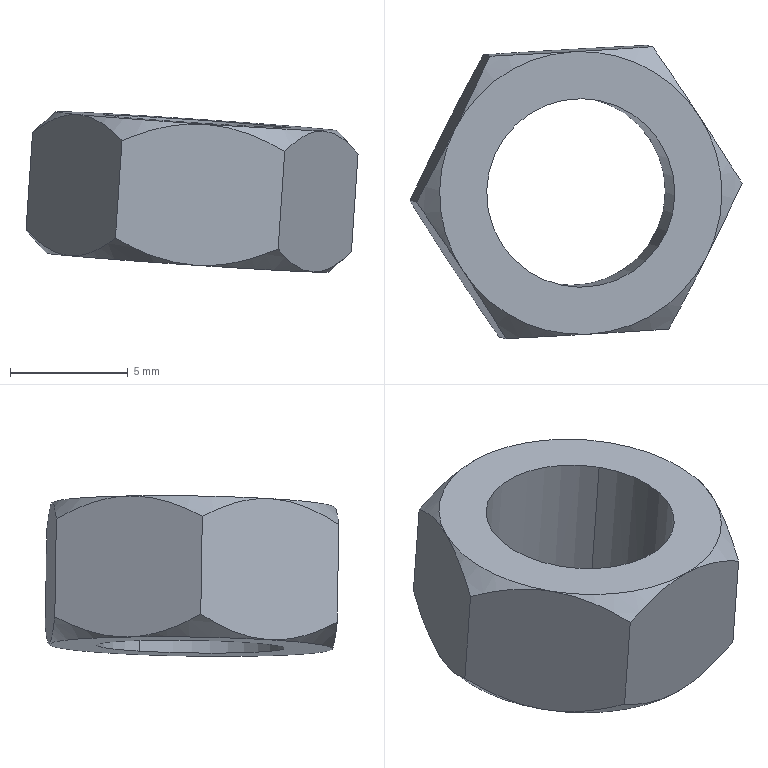Component | SolidWorks | SDAJ25x20-20B(00)+()-1_SDAJ-25- M8x1_25-1 | 1 solid | 22 faces | box 14.08 x 12.45 x 6.82 mm | volume 440 mm3 | cone 12 | plane 8 | cylinder 2 | commonest cylinder face diameters 8 x2
STEP:
#1=CARTESIAN_POINT('',(-3.493,5.702,30.763));
#2=VERTEX_POINT('',#1);
#3=CARTESIAN_POINT('',(-3.756,5.529,30.778));
#4=VERTEX_POINT('',#3);
#5=CARTESIAN_POINT('',(-3.493,5.702,30.763));
#6=CARTESIAN_POINT('',(-3.482,5.685,30.762));
#7=CARTESIAN_POINT('',(-3.474,5.666,30.761));
#8=CARTESIAN_POINT('',(-3.467,5.625,30.76));
#9=CARTESIAN_POINT('',(-3.467,5.604,30.76));
#10=CARTESIAN_POINT('',(-3.475,5.564,30.76));
#11=CARTESIAN_POINT('',(-3.483,5.544,30.76));
#12=CARTESIAN_POINT('',(-3.506,5.51,30.761));
#13=CARTESIAN_POINT('',(-3.521,5.495,30.762));
#14=CARTESIAN_POINT('',(-3.556,5.473,30.764));
#15=CARTESIAN_POINT('',(-3.575,5.465,30.765));
#16=CARTESIAN_POINT('',(-3.616,5.457,30.768));
#17=CARTESIAN_POINT('',(-3.636,5.457,30.769));
#18=CARTESIAN_POINT('',(-3.677,5.466,30.772));
#19=CARTESIAN_POINT('',(-3.696,5.474,30.773));
#20=CARTESIAN_POINT('',(-3.73,5.497,30.776));
#21=CARTESIAN_POINT('',(-3.745,5.512,30.777));
#22=CARTESIAN_POINT('',(-3.756,5.529,30.778));
#23=B_SPLINE_CURVE_WITH_KNOTS('',3,(#5,#6,#7,#8,#9,#10,#11,#12,#13,#14,#15,#16,#17,#18,#19,#20,#21,#22),.UNSPECIFIED.,.F.,.F.,(4,2,2,2,2,2,2,2,4),(0.,0.0625,0.125,0.1875,0.25,0.3125,0.375,0.4375,0.5),.UNSPECIFIED.);
#24=EDGE_CURVE('',#2,#4,#23,.T.);
#25=ORIENTED_EDGE('',*,*,#24,.F.);
#26=CARTESIAN_POINT('',(-3.509,5.706,30.527));
#27=VERTEX_POINT('',#26);
#28=CARTESIAN_POINT('',(-3.493,5.702,30.763));
#29=DIRECTION('',(-0.0675,0.01553,-0.9976));
#30=VECTOR('',#29,39.37);
#31=LINE('',#28,#30);
#32=EDGE_CURVE('',#2,#27,#31,.T.);
#33=ORIENTED_EDGE('',*,*,#32,.T.);
#34=CARTESIAN_POINT('',(-3.772,5.533,30.543));
#35=VERTEX_POINT('',#34);
#36=CARTESIAN_POINT('',(-3.641,5.619,30.535));
#37=DIRECTION('',(-0.0675,0.01553,-0.9976));
#38=DIRECTION('',(-0.8341,-0.5496,0.04788));
#39=AXIS2_PLACEMENT_3D('',#36,#37,#38);
#40=CIRCLE('',#39,0.1575);
#41=EDGE_CURVE('',#27,#35,#40,.T.);
#42=ORIENTED_EDGE('',*,*,#41,.T.);
#43=CARTESIAN_POINT('',(-3.756,5.529,30.778));
#44=DIRECTION('',(-0.0675,0.01553,-0.9976));
#45=VECTOR('',#44,39.37);
#46=LINE('',#43,#45);
#47=EDGE_CURVE('',#4,#35,#46,.T.);
#48=ORIENTED_EDGE('',*,*,#47,.F.);
#49=EDGE_LOOP('',(#25,#33,#42,#48));
#50=FACE_OUTER_BOUND('',#49,.T.);
#51=CARTESIAN_POINT('',(-3.625,5.616,30.771));
#52=DIRECTION('',(-0.0675,0.01553,-0.9976));
#53=DIRECTION('',(-0.8341,-0.5496,0.04788));
#54=AXIS2_PLACEMENT_3D('',#51,#52,#53);
#55=CYLINDRICAL_SURFACE('',#54,0.1575);
#56=ADVANCED_FACE('',(#50),#55,.F.);
#57=CARTESIAN_POINT('',(-3.611,5.38,30.766));
#58=VERTEX_POINT('',#57);
#59=CARTESIAN_POINT('',(-3.478,5.388,30.721));
#60=VERTEX_POINT('',#59);
#61=CARTESIAN_POINT('',(-3.611,5.38,30.766));
#62=CARTESIAN_POINT('',(-3.588,5.381,30.764));
#63=CARTESIAN_POINT('',(-3.565,5.383,30.759));
#64=CARTESIAN_POINT('',(-3.52,5.386,30.743));
#65=CARTESIAN_POINT('',(-3.498,5.387,30.733));
#66=CARTESIAN_POINT('',(-3.478,5.388,30.721));
#67=B_SPLINE_CURVE_WITH_KNOTS('',3,(#61,#62,#63,#64,#65,#66),.UNSPECIFIED.,.F.,.F.,(4,2,4),(0.003591,0.005374,0.007157),.UNSPECIFIED.);
#68=EDGE_CURVE('',#58,#60,#67,.T.);
#69=ORIENTED_EDGE('',*,*,#68,.T.);
#70=CARTESIAN_POINT('',(-3.414,5.51,30.755));
#71=VERTEX_POINT('',#70);
#72=CARTESIAN_POINT('',(-3.478,5.388,30.721));
#73=CARTESIAN_POINT('',(-3.468,5.407,30.731));
#74=CARTESIAN_POINT('',(-3.457,5.427,30.74));
#75=CARTESIAN_POINT('',(-3.441,5.457,30.749));
#76=CARTESIAN_POINT('',(-3.436,5.467,30.751));
#77=CARTESIAN_POINT('',(-3.425,5.488,30.754));
#78=CARTESIAN_POINT('',(-3.42,5.499,30.755));
#79=CARTESIAN_POINT('',(-3.414,5.51,30.755));
#80=B_SPLINE_CURVE_WITH_KNOTS('',3,(#72,#73,#74,#75,#76,#77,#78,#79),.UNSPECIFIED.,.F.,.F.,(4,2,2,4),(0.00000025,0.001796,0.002693,0.003591),.UNSPECIFIED.);
#81=EDGE_CURVE('',#60,#71,#80,.T.);
#82=ORIENTED_EDGE('',*,*,#81,.T.);
#83=CARTESIAN_POINT('',(-3.625,5.616,30.771));
#84=DIRECTION('',(0.0675,-0.01553,0.9976));
#85=DIRECTION('',(0.8341,0.5496,-0.04788));
#86=AXIS2_PLACEMENT_3D('',#83,#84,#85);
#87=CIRCLE('',#86,0.2362);
#88=EDGE_CURVE('',#58,#71,#87,.T.);
#89=ORIENTED_EDGE('',*,*,#88,.F.);
#90=EDGE_LOOP('',(#69,#82,#89));
#91=FACE_OUTER_BOUND('',#90,.T.);
#92=CARTESIAN_POINT('',(-3.628,5.616,30.724));
#93=DIRECTION('',(-0.0675,0.01553,-0.9976));
#94=DIRECTION('',(-0.8341,-0.5496,0.04788));
#95=AXIS2_PLACEMENT_3D('',#92,#93,#94);
#96=CONICAL_SURFACE('',#95,0.2835,0.7854);
#97=ADVANCED_FACE('',(#91),#96,.T.);
#98=CARTESIAN_POINT('',(-3.428,5.745,30.759));
#99=VERTEX_POINT('',#98);
#100=CARTESIAN_POINT('',(-3.625,5.616,30.771));
#101=DIRECTION('',(0.0675,-0.01553,0.9976));
#102=DIRECTION('',(0.8341,0.5496,-0.04788));
#103=AXIS2_PLACEMENT_3D('',#100,#101,#102);
#104=CIRCLE('',#103,0.2362);
#105=EDGE_CURVE('',#71,#99,#104,.T.);
#106=ORIENTED_EDGE('',*,*,#105,.F.);
#107=CARTESIAN_POINT('',(-3.355,5.632,30.716));
#108=VERTEX_POINT('',#107);
#109=CARTESIAN_POINT('',(-3.414,5.51,30.755));
#110=CARTESIAN_POINT('',(-3.404,5.531,30.754));
#111=CARTESIAN_POINT('',(-3.393,5.552,30.75));
#112=CARTESIAN_POINT('',(-3.374,5.593,30.737));
#113=CARTESIAN_POINT('',(-3.364,5.613,30.727));
#114=CARTESIAN_POINT('',(-3.355,5.632,30.716));
#115=B_SPLINE_CURVE_WITH_KNOTS('',3,(#109,#110,#111,#112,#113,#114),.UNSPECIFIED.,.F.,.F.,(4,2,4),(0.003591,0.005374,0.007157),.UNSPECIFIED.);
#116=EDGE_CURVE('',#71,#108,#115,.T.);
#117=ORIENTED_EDGE('',*,*,#116,.T.);
#118=CARTESIAN_POINT('',(-3.355,5.632,30.716));
#119=CARTESIAN_POINT('',(-3.366,5.65,30.728));
#120=CARTESIAN_POINT('',(-3.378,5.668,30.738));
#121=CARTESIAN_POINT('',(-3.396,5.696,30.749));
#122=CARTESIAN_POINT('',(-3.402,5.706,30.753));
#123=CARTESIAN_POINT('',(-3.415,5.726,30.757));
#124=CARTESIAN_POINT('',(-3.421,5.735,30.759));
#125=CARTESIAN_POINT('',(-3.428,5.745,30.759));
#126=B_SPLINE_CURVE_WITH_KNOTS('',3,(#118,#119,#120,#121,#122,#123,#124,#125),.UNSPECIFIED.,.F.,.F.,(4,2,2,4),(0.004638,0.006433,0.007331,0.008228),.UNSPECIFIED.);
#127=EDGE_CURVE('',#108,#99,#126,.T.);
#128=ORIENTED_EDGE('',*,*,#127,.T.);
#129=EDGE_LOOP('',(#106,#117,#128));
#130=FACE_OUTER_BOUND('',#129,.T.);
#131=CARTESIAN_POINT('',(-3.628,5.616,30.724));
#132=DIRECTION('',(-0.0675,0.01553,-0.9976));
#133=DIRECTION('',(-0.8341,-0.5496,0.04788));
#134=AXIS2_PLACEMENT_3D('',#131,#132,#133);
#135=CONICAL_SURFACE('',#134,0.2835,0.7854);
#136=ADVANCED_FACE('',(#130),#135,.T.);
#137=CARTESIAN_POINT('',(-3.638,5.851,30.775));
#138=VERTEX_POINT('',#137);
#139=CARTESIAN_POINT('',(-3.625,5.616,30.771));
#140=DIRECTION('',(0.0675,-0.01553,0.9976));
#141=DIRECTION('',(0.8341,0.5496,-0.04788));
#142=AXIS2_PLACEMENT_3D('',#139,#140,#141);
#143=CIRCLE('',#142,0.2362);
#144=EDGE_CURVE('',#99,#138,#143,.T.);
#145=ORIENTED_EDGE('',*,*,#144,.F.);
#146=CARTESIAN_POINT('',(-3.505,5.86,30.73));
#147=VERTEX_POINT('',#146);
#148=CARTESIAN_POINT('',(-3.428,5.745,30.759));
#149=CARTESIAN_POINT('',(-3.441,5.766,30.761));
#150=CARTESIAN_POINT('',(-3.454,5.785,30.758));
#151=CARTESIAN_POINT('',(-3.473,5.814,30.75));
#152=CARTESIAN_POINT('',(-3.48,5.823,30.747));
#153=CARTESIAN_POINT('',(-3.492,5.842,30.739));
#154=CARTESIAN_POINT('',(-3.499,5.851,30.734));
#155=CARTESIAN_POINT('',(-3.505,5.86,30.73));
#156=B_SPLINE_CURVE_WITH_KNOTS('',3,(#148,#149,#150,#151,#152,#153,#154,#155),.UNSPECIFIED.,.F.,.F.,(4,2,2,4),(0.008228,0.01003,0.01092,0.01182),.UNSPECIFIED.);
#157=EDGE_CURVE('',#99,#147,#156,.T.);
#158=ORIENTED_EDGE('',*,*,#157,.T.);
#159=CARTESIAN_POINT('',(-3.505,5.86,30.73));
#160=CARTESIAN_POINT('',(-3.525,5.859,30.742));
#161=CARTESIAN_POINT('',(-3.547,5.857,30.752));
#162=CARTESIAN_POINT('',(-3.58,5.855,30.764));
#163=CARTESIAN_POINT('',(-3.591,5.854,30.768));
#164=CARTESIAN_POINT('',(-3.614,5.853,30.773));
#165=CARTESIAN_POINT('',(-3.626,5.852,30.774));
#166=CARTESIAN_POINT('',(-3.638,5.851,30.775));
#167=B_SPLINE_CURVE_WITH_KNOTS('',3,(#159,#160,#161,#162,#163,#164,#165,#166),.UNSPECIFIED.,.F.,.F.,(4,2,2,4),(0.00000025,0.001796,0.002693,0.003591),.UNSPECIFIED.);
#168=EDGE_CURVE('',#147,#138,#167,.T.);
#169=ORIENTED_EDGE('',*,*,#168,.T.);
#170=EDGE_LOOP('',(#145,#158,#169));
#171=FACE_OUTER_BOUND('',#170,.T.);
#172=CARTESIAN_POINT('',(-3.628,5.616,30.724));
#173=DIRECTION('',(-0.0675,0.01553,-0.9976));
#174=DIRECTION('',(-0.8341,-0.5496,0.04788));
#175=AXIS2_PLACEMENT_3D('',#172,#173,#174);
#176=CONICAL_SURFACE('',#175,0.2835,0.7854);
#177=ADVANCED_FACE('',(#171),#176,.T.);
#178=CARTESIAN_POINT('',(-3.822,5.486,30.782));
#179=VERTEX_POINT('',#178);
#180=CARTESIAN_POINT('',(-3.75,5.372,30.739));
#181=VERTEX_POINT('',#180);
#182=CARTESIAN_POINT('',(-3.822,5.486,30.782));
#183=CARTESIAN_POINT('',(-3.815,5.476,30.781));
#184=CARTESIAN_POINT('',(-3.809,5.466,30.78));
#185=CARTESIAN_POINT('',(-3.796,5.446,30.775));
#186=CARTESIAN_POINT('',(-3.79,5.437,30.772));
#187=CARTESIAN_POINT('',(-3.772,5.408,30.761));
#188=CARTESIAN_POINT('',(-3.76,5.39,30.75));
#189=CARTESIAN_POINT('',(-3.75,5.372,30.739));
#190=B_SPLINE_CURVE_WITH_KNOTS('',3,(#182,#183,#184,#185,#186,#187,#188,#189),.UNSPECIFIED.,.F.,.F.,(4,2,2,4),(0.007255,0.008152,0.009049,0.01084),.UNSPECIFIED.);
#191=EDGE_CURVE('',#179,#181,#190,.T.);
#192=ORIENTED_EDGE('',*,*,#191,.T.);
#193=CARTESIAN_POINT('',(-3.75,5.372,30.739));
#194=CARTESIAN_POINT('',(-3.728,5.374,30.748));
#195=CARTESIAN_POINT('',(-3.705,5.375,30.756));
#196=CARTESIAN_POINT('',(-3.671,5.377,30.763));
#197=CARTESIAN_POINT('',(-3.659,5.377,30.765));
#198=CARTESIAN_POINT('',(-3.635,5.378,30.767));
#199=CARTESIAN_POINT('',(-3.623,5.379,30.767));
#200=CARTESIAN_POINT('',(-3.611,5.38,30.766));
#201=B_SPLINE_CURVE_WITH_KNOTS('',3,(#193,#194,#195,#196,#197,#198,#199,#200),.UNSPECIFIED.,.F.,.F.,(4,2,2,4),(0.00000025,0.001796,0.002693,0.003591),.UNSPECIFIED.);
#202=EDGE_CURVE('',#181,#58,#201,.T.);
#203=ORIENTED_EDGE('',*,*,#202,.T.);
#204=CARTESIAN_POINT('',(-3.625,5.616,30.771));
#205=DIRECTION('',(0.0675,-0.01553,0.9976));
#206=DIRECTION('',(0.8341,0.5496,-0.04788));
#207=AXIS2_PLACEMENT_3D('',#204,#205,#206);
#208=CIRCLE('',#207,0.2362);
#209=EDGE_CURVE('',#179,#58,#208,.T.);
#210=ORIENTED_EDGE('',*,*,#209,.F.);
#211=EDGE_LOOP('',(#192,#203,#210));
#212=FACE_OUTER_BOUND('',#211,.T.);
#213=CARTESIAN_POINT('',(-3.628,5.616,30.724));
#214=DIRECTION('',(-0.0675,0.01553,-0.9976));
#215=DIRECTION('',(-0.8341,-0.5496,0.04788));
#216=AXIS2_PLACEMENT_3D('',#213,#214,#215);
#217=CONICAL_SURFACE('',#216,0.2835,0.7854);
#218=ADVANCED_FACE('',(#212),#217,.T.);
#219=CARTESIAN_POINT('',(-3.835,5.722,30.787));
#220=VERTEX_POINT('',#219);
#221=CARTESIAN_POINT('',(-3.625,5.616,30.771));
#222=DIRECTION('',(0.0675,-0.01553,0.9976));
#223=DIRECTION('',(0.8341,0.5496,-0.04788));
#224=AXIS2_PLACEMENT_3D('',#221,#222,#223);
#225=CIRCLE('',#224,0.2362);
#226=EDGE_CURVE('',#138,#220,#225,.T.);
#227=ORIENTED_EDGE('',*,*,#226,.F.);
#228=CARTESIAN_POINT('',(-3.777,5.844,30.748));
#229=VERTEX_POINT('',#228);
#230=CARTESIAN_POINT('',(-3.638,5.851,30.775));
#231=CARTESIAN_POINT('',(-3.662,5.85,30.777));
#232=CARTESIAN_POINT('',(-3.685,5.849,30.775));
#233=CARTESIAN_POINT('',(-3.732,5.846,30.765));
#234=CARTESIAN_POINT('',(-3.755,5.845,30.757));
#235=CARTESIAN_POINT('',(-3.777,5.844,30.748));
#236=B_SPLINE_CURVE_WITH_KNOTS('',3,(#230,#231,#232,#233,#234,#235),.UNSPECIFIED.,.F.,.F.,(4,2,4),(0.003591,0.005374,0.007157),.UNSPECIFIED.);
#237=EDGE_CURVE('',#138,#229,#236,.T.);
#238=ORIENTED_EDGE('',*,*,#237,.T.);
#239=CARTESIAN_POINT('',(-3.777,5.844,30.748));
#240=CARTESIAN_POINT('',(-3.785,5.825,30.759));
#241=CARTESIAN_POINT('',(-3.795,5.805,30.768));
#242=CARTESIAN_POINT('',(-3.809,5.775,30.779));
#243=CARTESIAN_POINT('',(-3.814,5.764,30.781));
#244=CARTESIAN_POINT('',(-3.824,5.743,30.785));
#245=CARTESIAN_POINT('',(-3.83,5.732,30.786));
#246=CARTESIAN_POINT('',(-3.835,5.722,30.787));
#247=B_SPLINE_CURVE_WITH_KNOTS('',3,(#239,#240,#241,#242,#243,#244,#245,#246),.UNSPECIFIED.,.F.,.F.,(4,2,2,4),(0.00000025,0.001796,0.002693,0.003591),.UNSPECIFIED.);
#248=EDGE_CURVE('',#229,#220,#247,.T.);
#249=ORIENTED_EDGE('',*,*,#248,.T.);
#250=EDGE_LOOP('',(#227,#238,#249));
#251=FACE_OUTER_BOUND('',#250,.T.);
#252=CARTESIAN_POINT('',(-3.628,5.616,30.724));
#253=DIRECTION('',(-0.0675,0.01553,-0.9976));
#254=DIRECTION('',(-0.8341,-0.5496,0.04788));
#255=AXIS2_PLACEMENT_3D('',#252,#253,#254);
#256=CONICAL_SURFACE('',#255,0.2835,0.7854);
#257=ADVANCED_FACE('',(#251),#256,.T.);
#258=CARTESIAN_POINT('',(-3.851,5.725,30.551));
#259=VERTEX_POINT('',#258);
#260=CARTESIAN_POINT('',(-3.788,5.847,30.585));
#261=VERTEX_POINT('',#260);
#262=CARTESIAN_POINT('',(-3.851,5.725,30.551));
#263=CARTESIAN_POINT('',(-3.841,5.747,30.55));
#264=CARTESIAN_POINT('',(-3.83,5.767,30.554));
#265=CARTESIAN_POINT('',(-3.808,5.808,30.566));
#266=CARTESIAN_POINT('',(-3.798,5.828,30.575));
#267=CARTESIAN_POINT('',(-3.788,5.847,30.585));
#268=B_SPLINE_CURVE_WITH_KNOTS('',3,(#262,#263,#264,#265,#266,#267),.UNSPECIFIED.,.F.,.F.,(4,2,4),(0.003591,0.005374,0.007157),.UNSPECIFIED.);
#269=EDGE_CURVE('',#259,#261,#268,.T.);
#270=ORIENTED_EDGE('',*,*,#269,.T.);
#271=CARTESIAN_POINT('',(-3.654,5.855,30.54));
#272=VERTEX_POINT('',#271);
#273=CARTESIAN_POINT('',(-3.788,5.847,30.585));
#274=CARTESIAN_POINT('',(-3.767,5.848,30.573));
#275=CARTESIAN_POINT('',(-3.746,5.849,30.562));
#276=CARTESIAN_POINT('',(-3.713,5.852,30.551));
#277=CARTESIAN_POINT('',(-3.701,5.852,30.547));
#278=CARTESIAN_POINT('',(-3.678,5.854,30.542));
#279=CARTESIAN_POINT('',(-3.666,5.854,30.54));
#280=CARTESIAN_POINT('',(-3.654,5.855,30.54));
#281=B_SPLINE_CURVE_WITH_KNOTS('',3,(#273,#274,#275,#276,#277,#278,#279,#280),.UNSPECIFIED.,.F.,.F.,(4,2,2,4),(0.00000025,0.001796,0.002693,0.003591),.UNSPECIFIED.);
#282=EDGE_CURVE('',#261,#272,#281,.T.);
#283=ORIENTED_EDGE('',*,*,#282,.T.);
#284=CARTESIAN_POINT('',(-3.641,5.619,30.535));
#285=DIRECTION('',(0.0675,-0.01553,0.9976));
#286=DIRECTION('',(0.8341,0.5496,-0.04788));
#287=AXIS2_PLACEMENT_3D('',#284,#285,#286);
#288=CIRCLE('',#287,0.2362);
#289=EDGE_CURVE('',#272,#259,#288,.T.);
#290=ORIENTED_EDGE('',*,*,#289,.T.);
#291=EDGE_LOOP('',(#270,#283,#290));
#292=FACE_OUTER_BOUND('',#291,.T.);
#293=CARTESIAN_POINT('',(-3.641,5.619,30.535));
#294=DIRECTION('',(0.0675,-0.01553,0.9976));
#295=DIRECTION('',(0.8341,0.5496,-0.04788));
#296=AXIS2_PLACEMENT_3D('',#293,#294,#295);
#297=CONICAL_SURFACE('',#296,0.2362,0.7854);
#298=ADVANCED_FACE('',(#292),#297,.T.);
#299=CARTESIAN_POINT('',(-3.444,5.749,30.524));
#300=VERTEX_POINT('',#299);
#301=CARTESIAN_POINT('',(-3.641,5.619,30.535));
#302=DIRECTION('',(0.0675,-0.01553,0.9976));
#303=DIRECTION('',(0.8341,0.5496,-0.04788));
#304=AXIS2_PLACEMENT_3D('',#301,#302,#303);
#305=CIRCLE('',#304,0.2362);
#306=EDGE_CURVE('',#300,#272,#305,.T.);
#307=ORIENTED_EDGE('',*,*,#306,.T.);
#308=CARTESIAN_POINT('',(-3.516,5.863,30.567));
#309=VERTEX_POINT('',#308);
#310=CARTESIAN_POINT('',(-3.654,5.855,30.54));
#311=CARTESIAN_POINT('',(-3.631,5.857,30.538));
#312=CARTESIAN_POINT('',(-3.607,5.858,30.54));
#313=CARTESIAN_POINT('',(-3.56,5.86,30.55));
#314=CARTESIAN_POINT('',(-3.538,5.861,30.558));
#315=CARTESIAN_POINT('',(-3.516,5.863,30.567));
#316=B_SPLINE_CURVE_WITH_KNOTS('',3,(#310,#311,#312,#313,#314,#315),.UNSPECIFIED.,.F.,.F.,(4,2,4),(0.003591,0.005374,0.007157),.UNSPECIFIED.);
#317=EDGE_CURVE('',#272,#309,#316,.T.);
#318=ORIENTED_EDGE('',*,*,#317,.T.);
#319=CARTESIAN_POINT('',(-3.516,5.863,30.567));
#320=CARTESIAN_POINT('',(-3.51,5.854,30.561));
#321=CARTESIAN_POINT('',(-3.505,5.845,30.556));
#322=CARTESIAN_POINT('',(-3.493,5.827,30.546));
#323=CARTESIAN_POINT('',(-3.487,5.817,30.541));
#324=CARTESIAN_POINT('',(-3.469,5.789,30.53));
#325=CARTESIAN_POINT('',(-3.457,5.769,30.525));
#326=CARTESIAN_POINT('',(-3.444,5.749,30.524));
#327=B_SPLINE_CURVE_WITH_KNOTS('',3,(#319,#320,#321,#322,#323,#324,#325,#326),.UNSPECIFIED.,.F.,.F.,(4,2,2,4),(0.003664,0.004562,0.00546,0.007255),.UNSPECIFIED.);
#328=EDGE_CURVE('',#309,#300,#327,.T.);
#329=ORIENTED_EDGE('',*,*,#328,.T.);
#330=EDGE_LOOP('',(#307,#318,#329));
#331=FACE_OUTER_BOUND('',#330,.T.);
#332=CARTESIAN_POINT('',(-3.641,5.619,30.535));
#333=DIRECTION('',(0.0675,-0.01553,0.9976));
#334=DIRECTION('',(0.8341,0.5496,-0.04788));
#335=AXIS2_PLACEMENT_3D('',#332,#333,#334);
#336=CONICAL_SURFACE('',#335,0.2362,0.7854);
#337=ADVANCED_FACE('',(#331),#336,.T.);
#338=CARTESIAN_POINT('',(-3.43,5.513,30.519));
#339=VERTEX_POINT('',#338);
#340=CARTESIAN_POINT('',(-3.641,5.619,30.535));
#341=DIRECTION('',(0.0675,-0.01553,0.9976));
#342=DIRECTION('',(0.8341,0.5496,-0.04788));
#343=AXIS2_PLACEMENT_3D('',#340,#341,#342);
#344=CIRCLE('',#343,0.2362);
#345=EDGE_CURVE('',#339,#300,#344,.T.);
#346=ORIENTED_EDGE('',*,*,#345,.T.);
#347=CARTESIAN_POINT('',(-3.366,5.635,30.553));
#348=VERTEX_POINT('',#347);
#349=CARTESIAN_POINT('',(-3.444,5.749,30.524));
#350=CARTESIAN_POINT('',(-3.437,5.739,30.523));
#351=CARTESIAN_POINT('',(-3.43,5.729,30.523));
#352=CARTESIAN_POINT('',(-3.417,5.71,30.526));
#353=CARTESIAN_POINT('',(-3.411,5.7,30.528));
#354=CARTESIAN_POINT('',(-3.392,5.671,30.536));
#355=CARTESIAN_POINT('',(-3.379,5.653,30.544));
#356=CARTESIAN_POINT('',(-3.366,5.635,30.553));
#357=B_SPLINE_CURVE_WITH_KNOTS('',3,(#349,#350,#351,#352,#353,#354,#355,#356),.UNSPECIFIED.,.F.,.F.,(4,2,2,4),(0.007255,0.008152,0.009049,0.01084),.UNSPECIFIED.);
#358=EDGE_CURVE('',#300,#348,#357,.T.);
#359=ORIENTED_EDGE('',*,*,#358,.T.);
#360=CARTESIAN_POINT('',(-3.366,5.635,30.553));
#361=CARTESIAN_POINT('',(-3.377,5.616,30.543));
#362=CARTESIAN_POINT('',(-3.387,5.596,30.534));
#363=CARTESIAN_POINT('',(-3.403,5.566,30.525));
#364=CARTESIAN_POINT('',(-3.408,5.556,30.523));
#365=CARTESIAN_POINT('',(-3.419,5.535,30.52));
#366=CARTESIAN_POINT('',(-3.425,5.524,30.519));
#367=CARTESIAN_POINT('',(-3.43,5.513,30.519));
#368=B_SPLINE_CURVE_WITH_KNOTS('',3,(#360,#361,#362,#363,#364,#365,#366,#367),.UNSPECIFIED.,.F.,.F.,(4,2,2,4),(0.00000025,0.001796,0.002693,0.003591),.UNSPECIFIED.);
#369=EDGE_CURVE('',#348,#339,#368,.T.);
#370=ORIENTED_EDGE('',*,*,#369,.T.);
#371=EDGE_LOOP('',(#346,#359,#370));
#372=FACE_OUTER_BOUND('',#371,.T.);
#373=CARTESIAN_POINT('',(-3.641,5.619,30.535));
#374=DIRECTION('',(0.0675,-0.01553,0.9976));
#375=DIRECTION('',(0.8341,0.5496,-0.04788));
#376=AXIS2_PLACEMENT_3D('',#373,#374,#375);
#377=CONICAL_SURFACE('',#376,0.2362,0.7854);
#378=ADVANCED_FACE('',(#372),#377,.T.);
#379=CARTESIAN_POINT('',(-3.627,5.384,30.53));
#380=VERTEX_POINT('',#379);
#381=CARTESIAN_POINT('',(-3.641,5.619,30.535));
#382=DIRECTION('',(0.0675,-0.01553,0.9976));
#383=DIRECTION('',(0.8341,0.5496,-0.04788));
#384=AXIS2_PLACEMENT_3D('',#381,#382,#383);
#385=CIRCLE('',#384,0.2362);
#386=EDGE_CURVE('',#380,#339,#385,.T.);
#387=ORIENTED_EDGE('',*,*,#386,.T.);
#388=CARTESIAN_POINT('',(-3.489,5.391,30.558));
#389=VERTEX_POINT('',#388);
#390=CARTESIAN_POINT('',(-3.43,5.513,30.519));
#391=CARTESIAN_POINT('',(-3.441,5.492,30.519));
#392=CARTESIAN_POINT('',(-3.451,5.471,30.523));
#393=CARTESIAN_POINT('',(-3.471,5.43,30.537));
#394=CARTESIAN_POINT('',(-3.48,5.41,30.547));
#395=CARTESIAN_POINT('',(-3.489,5.391,30.558));
#396=B_SPLINE_CURVE_WITH_KNOTS('',3,(#390,#391,#392,#393,#394,#395),.UNSPECIFIED.,.F.,.F.,(4,2,4),(0.003591,0.005374,0.007157),.UNSPECIFIED.);
#397=EDGE_CURVE('',#339,#389,#396,.T.);
#398=ORIENTED_EDGE('',*,*,#397,.T.);
#399=CARTESIAN_POINT('',(-3.489,5.391,30.558));
#400=CARTESIAN_POINT('',(-3.511,5.39,30.549));
#401=CARTESIAN_POINT('',(-3.533,5.389,30.541));
#402=CARTESIAN_POINT('',(-3.568,5.387,30.533));
#403=CARTESIAN_POINT('',(-3.579,5.386,30.532));
#404=CARTESIAN_POINT('',(-3.603,5.385,30.53));
#405=CARTESIAN_POINT('',(-3.615,5.384,30.53));
#406=CARTESIAN_POINT('',(-3.627,5.384,30.53));
#407=B_SPLINE_CURVE_WITH_KNOTS('',3,(#399,#400,#401,#402,#403,#404,#405,#406),.UNSPECIFIED.,.F.,.F.,(4,2,2,4),(0.00000025,0.001796,0.002693,0.003591),.UNSPECIFIED.);
#408=EDGE_CURVE('',#389,#380,#407,.T.);
#409=ORIENTED_EDGE('',*,*,#408,.T.);
#410=EDGE_LOOP('',(#387,#398,#409));
#411=FACE_OUTER_BOUND('',#410,.T.);
#412=CARTESIAN_POINT('',(-3.641,5.619,30.535));
#413=DIRECTION('',(0.0675,-0.01553,0.9976));
#414=DIRECTION('',(0.8341,0.5496,-0.04788));
#415=AXIS2_PLACEMENT_3D('',#412,#413,#414);
#416=CONICAL_SURFACE('',#415,0.2362,0.7854);
#417=ADVANCED_FACE('',(#411),#416,.T.);
#418=CARTESIAN_POINT('',(-3.838,5.49,30.546));
#419=VERTEX_POINT('',#418);
#420=CARTESIAN_POINT('',(-3.641,5.619,30.535));
#421=DIRECTION('',(0.0675,-0.01553,0.9976));
#422=DIRECTION('',(0.8341,0.5496,-0.04788));
#423=AXIS2_PLACEMENT_3D('',#420,#421,#422);
#424=CIRCLE('',#423,0.2362);
#425=EDGE_CURVE('',#419,#380,#424,.T.);
#426=ORIENTED_EDGE('',*,*,#425,.T.);
#427=CARTESIAN_POINT('',(-3.761,5.375,30.576));
#428=VERTEX_POINT('',#427);
#429=CARTESIAN_POINT('',(-3.627,5.384,30.53));
#430=CARTESIAN_POINT('',(-3.651,5.382,30.532));
#431=CARTESIAN_POINT('',(-3.674,5.381,30.537));
#432=CARTESIAN_POINT('',(-3.719,5.378,30.553));
#433=CARTESIAN_POINT('',(-3.74,5.376,30.564));
#434=CARTESIAN_POINT('',(-3.761,5.375,30.576));
#435=B_SPLINE_CURVE_WITH_KNOTS('',3,(#429,#430,#431,#432,#433,#434),.UNSPECIFIED.,.F.,.F.,(4,2,4),(0.003591,0.005374,0.007157),.UNSPECIFIED.);
#436=EDGE_CURVE('',#380,#428,#435,.T.);
#437=ORIENTED_EDGE('',*,*,#436,.T.);
#438=CARTESIAN_POINT('',(-3.761,5.375,30.576));
#439=CARTESIAN_POINT('',(-3.773,5.393,30.566));
#440=CARTESIAN_POINT('',(-3.786,5.412,30.558));
#441=CARTESIAN_POINT('',(-3.805,5.44,30.55));
#442=CARTESIAN_POINT('',(-3.811,5.45,30.548));
#443=CARTESIAN_POINT('',(-3.825,5.47,30.546));
#444=CARTESIAN_POINT('',(-3.831,5.48,30.546));
#445=CARTESIAN_POINT('',(-3.838,5.49,30.546));
#446=B_SPLINE_CURVE_WITH_KNOTS('',3,(#438,#439,#440,#441,#442,#443,#444,#445),.UNSPECIFIED.,.F.,.F.,(4,2,2,4),(0.004638,0.006433,0.007331,0.008228),.UNSPECIFIED.);
#447=EDGE_CURVE('',#428,#419,#446,.T.);
#448=ORIENTED_EDGE('',*,*,#447,.T.);
#449=EDGE_LOOP('',(#426,#437,#448));
#450=FACE_OUTER_BOUND('',#449,.T.);
#451=CARTESIAN_POINT('',(-3.641,5.619,30.535));
#452=DIRECTION('',(0.0675,-0.01553,0.9976));
#453=DIRECTION('',(0.8341,0.5496,-0.04788));
#454=AXIS2_PLACEMENT_3D('',#451,#452,#453);
#455=CONICAL_SURFACE('',#454,0.2362,0.7854);
#456=ADVANCED_FACE('',(#450),#455,.T.);
#457=ORIENTED_EDGE('',*,*,#144,.T.);
#458=ORIENTED_EDGE('',*,*,#226,.T.);
#459=CARTESIAN_POINT('',(-3.625,5.616,30.771));
#460=DIRECTION('',(0.0675,-0.01553,0.9976));
#461=DIRECTION('',(0.8341,0.5496,-0.04788));
#462=AXIS2_PLACEMENT_3D('',#459,#460,#461);
#463=CIRCLE('',#462,0.2362);
#464=EDGE_CURVE('',#220,#179,#463,.T.);
#465=ORIENTED_EDGE('',*,*,#464,.T.);
#466=ORIENTED_EDGE('',*,*,#209,.T.);
#467=ORIENTED_EDGE('',*,*,#88,.T.);
#468=ORIENTED_EDGE('',*,*,#105,.T.);
#469=EDGE_LOOP('',(#457,#458,#465,#466,#467,#468));
#470=FACE_OUTER_BOUND('',#469,.T.);
#471=CARTESIAN_POINT('',(-3.756,5.529,30.778));
#472=CARTESIAN_POINT('',(-3.767,5.546,30.779));
#473=CARTESIAN_POINT('',(-3.775,5.566,30.78));
#474=CARTESIAN_POINT('',(-3.783,5.606,30.781));
#475=CARTESIAN_POINT('',(-3.783,5.627,30.782));
#476=CARTESIAN_POINT('',(-3.774,5.668,30.782));
#477=CARTESIAN_POINT('',(-3.766,5.687,30.781));
#478=CARTESIAN_POINT('',(-3.743,5.721,30.78));
#479=CARTESIAN_POINT('',(-3.728,5.736,30.78));
#480=CARTESIAN_POINT('',(-3.694,5.759,30.778));
#481=CARTESIAN_POINT('',(-3.674,5.766,30.776));
#482=CARTESIAN_POINT('',(-3.634,5.774,30.774));
#483=CARTESIAN_POINT('',(-3.613,5.774,30.772));
#484=CARTESIAN_POINT('',(-3.573,5.766,30.769));
#485=CARTESIAN_POINT('',(-3.553,5.758,30.768));
#486=CARTESIAN_POINT('',(-3.519,5.734,30.765));
#487=CARTESIAN_POINT('',(-3.505,5.72,30.764));
#488=CARTESIAN_POINT('',(-3.493,5.702,30.763));
#489=B_SPLINE_CURVE_WITH_KNOTS('',3,(#471,#472,#473,#474,#475,#476,#477,#478,#479,#480,#481,#482,#483,#484,#485,#486,#487,#488),.UNSPECIFIED.,.F.,.F.,(4,2,2,2,2,2,2,2,4),(0.5,0.5625,0.625,0.6875,0.75,0.8125,0.875,0.9375,1.),.UNSPECIFIED.);
#490=EDGE_CURVE('',#4,#2,#489,.T.);
#491=ORIENTED_EDGE('',*,*,#490,.T.);
#492=ORIENTED_EDGE('',*,*,#24,.T.);
#493=EDGE_LOOP('',(#491,#492));
#494=FACE_BOUND('',#493,.T.);
#495=CARTESIAN_POINT('',(-3.625,5.616,30.771));
#496=DIRECTION('',(-0.0675,0.01553,-0.9976));
#497=DIRECTION('',(-0.8341,-0.5496,0.04788));
#498=AXIS2_PLACEMENT_3D('',#495,#496,#497);
#499=PLANE('',#498);
#500=ADVANCED_FACE('',(#470,#494),#499,.F.);
#501=ORIENTED_EDGE('',*,*,#306,.F.);
#502=ORIENTED_EDGE('',*,*,#345,.F.);
#503=ORIENTED_EDGE('',*,*,#386,.F.);
#504=ORIENTED_EDGE('',*,*,#425,.F.);
#505=CARTESIAN_POINT('',(-3.641,5.619,30.535));
#506=DIRECTION('',(0.0675,-0.01553,0.9976));
#507=DIRECTION('',(0.8341,0.5496,-0.04788));
#508=AXIS2_PLACEMENT_3D('',#505,#506,#507);
#509=CIRCLE('',#508,0.2362);
#510=EDGE_CURVE('',#259,#419,#509,.T.);
#511=ORIENTED_EDGE('',*,*,#510,.F.);
#512=ORIENTED_EDGE('',*,*,#289,.F.);
#513=EDGE_LOOP('',(#501,#502,#503,#504,#511,#512));
#514=FACE_OUTER_BOUND('',#513,.T.);
#515=CARTESIAN_POINT('',(-3.641,5.619,30.535));
#516=DIRECTION('',(-0.0675,0.01553,-0.9976));
#517=DIRECTION('',(-0.8341,-0.5496,0.04788));
#518=AXIS2_PLACEMENT_3D('',#515,#516,#517);
#519=CIRCLE('',#518,0.1575);
#520=EDGE_CURVE('',#35,#27,#519,.T.);
#521=ORIENTED_EDGE('',*,*,#520,.F.);
#522=ORIENTED_EDGE('',*,*,#41,.F.);
#523=EDGE_LOOP('',(#521,#522));
#524=FACE_BOUND('',#523,.T.);
#525=CARTESIAN_POINT('',(-3.77,5.817,30.547));
#526=DIRECTION('',(0.0675,-0.01553,0.9976));
#527=DIRECTION('',(0.8341,0.5496,-0.04788));
#528=AXIS2_PLACEMENT_3D('',#525,#526,#527);
#529=PLANE('',#528);
#530=ADVANCED_FACE('',(#514,#524),#529,.F.);
#531=CARTESIAN_POINT('',(-3.899,5.6,30.752));
#532=VERTEX_POINT('',#531);
#533=CARTESIAN_POINT('',(-3.835,5.722,30.787));
#534=CARTESIAN_POINT('',(-3.846,5.7,30.787));
#535=CARTESIAN_POINT('',(-3.857,5.68,30.784));
#536=CARTESIAN_POINT('',(-3.878,5.639,30.771));
#537=CARTESIAN_POINT('',(-3.889,5.619,30.763));
#538=CARTESIAN_POINT('',(-3.899,5.6,30.752));
#539=B_SPLINE_CURVE_WITH_KNOTS('',3,(#533,#534,#535,#536,#537,#538),.UNSPECIFIED.,.F.,.F.,(4,2,4),(0.003591,0.005374,0.007157),.UNSPECIFIED.);
#540=EDGE_CURVE('',#220,#532,#539,.T.);
#541=ORIENTED_EDGE('',*,*,#540,.T.);
#542=CARTESIAN_POINT('',(-3.899,5.6,30.752));
#543=CARTESIAN_POINT('',(-3.893,5.591,30.757));
#544=CARTESIAN_POINT('',(-3.887,5.582,30.761));
#545=CARTESIAN_POINT('',(-3.874,5.564,30.769));
#546=CARTESIAN_POINT('',(-3.867,5.554,30.773));
#547=CARTESIAN_POINT('',(-3.848,5.525,30.781));
#548=CARTESIAN_POINT('',(-3.835,5.506,30.783));
#549=CARTESIAN_POINT('',(-3.822,5.486,30.782));
#550=B_SPLINE_CURVE_WITH_KNOTS('',3,(#542,#543,#544,#545,#546,#547,#548,#549),.UNSPECIFIED.,.F.,.F.,(4,2,2,4),(0.003664,0.004562,0.00546,0.007255),.UNSPECIFIED.);
#551=EDGE_CURVE('',#532,#179,#550,.T.);
#552=ORIENTED_EDGE('',*,*,#551,.T.);
#553=ORIENTED_EDGE('',*,*,#464,.F.);
#554=EDGE_LOOP('',(#541,#552,#553));
#555=FACE_OUTER_BOUND('',#554,.T.);
#556=CARTESIAN_POINT('',(-3.628,5.616,30.724));
#557=DIRECTION('',(-0.0675,0.01553,-0.9976));
#558=DIRECTION('',(-0.8341,-0.5496,0.04788));
#559=AXIS2_PLACEMENT_3D('',#556,#557,#558);
#560=CONICAL_SURFACE('',#559,0.2835,0.7854);
#561=ADVANCED_FACE('',(#555),#560,.T.);
#562=ORIENTED_EDGE('',*,*,#510,.T.);
#563=CARTESIAN_POINT('',(-3.91,5.603,30.59));
#564=VERTEX_POINT('',#563);
#565=CARTESIAN_POINT('',(-3.838,5.49,30.546));
#566=CARTESIAN_POINT('',(-3.851,5.51,30.547));
#567=CARTESIAN_POINT('',(-3.863,5.529,30.552));
#568=CARTESIAN_POINT('',(-3.881,5.557,30.564));
#569=CARTESIAN_POINT('',(-3.887,5.567,30.568));
#570=CARTESIAN_POINT('',(-3.899,5.585,30.578));
#571=CARTESIAN_POINT('',(-3.904,5.594,30.584));
#572=CARTESIAN_POINT('',(-3.91,5.603,30.59));
#573=B_SPLINE_CURVE_WITH_KNOTS('',3,(#565,#566,#567,#568,#569,#570,#571,#572),.UNSPECIFIED.,.F.,.F.,(4,2,2,4),(0.008228,0.01003,0.01092,0.01182),.UNSPECIFIED.);
#574=EDGE_CURVE('',#419,#564,#573,.T.);
#575=ORIENTED_EDGE('',*,*,#574,.T.);
#576=CARTESIAN_POINT('',(-3.91,5.603,30.59));
#577=CARTESIAN_POINT('',(-3.901,5.622,30.579));
#578=CARTESIAN_POINT('',(-3.892,5.642,30.569));
#579=CARTESIAN_POINT('',(-3.877,5.672,30.559));
#580=CARTESIAN_POINT('',(-3.872,5.683,30.556));
#581=CARTESIAN_POINT('',(-3.862,5.704,30.552));
#582=CARTESIAN_POINT('',(-3.857,5.715,30.551));
#583=CARTESIAN_POINT('',(-3.851,5.725,30.551));
#584=B_SPLINE_CURVE_WITH_KNOTS('',3,(#576,#577,#578,#579,#580,#581,#582,#583),.UNSPECIFIED.,.F.,.F.,(4,2,2,4),(0.00000025,0.001796,0.002693,0.003591),.UNSPECIFIED.);
#585=EDGE_CURVE('',#564,#259,#584,.T.);
#586=ORIENTED_EDGE('',*,*,#585,.T.);
#587=EDGE_LOOP('',(#562,#575,#586));
#588=FACE_OUTER_BOUND('',#587,.T.);
#589=CARTESIAN_POINT('',(-3.641,5.619,30.535));
#590=DIRECTION('',(0.0675,-0.01553,0.9976));
#591=DIRECTION('',(0.8341,0.5496,-0.04788));
#592=AXIS2_PLACEMENT_3D('',#589,#590,#591);
#593=CONICAL_SURFACE('',#592,0.2362,0.7854);
#594=ADVANCED_FACE('',(#588),#593,.T.);
#595=CARTESIAN_POINT('',(-3.566,5.874,29.824));
#596=DIRECTION('',(0.0675,-0.01553,0.9976));
#597=VECTOR('',#596,39.37);
#598=LINE('',#595,#597);
#599=EDGE_CURVE('',#309,#147,#598,.T.);
#600=ORIENTED_EDGE('',*,*,#599,.F.);
#601=ORIENTED_EDGE('',*,*,#317,.F.);
#602=ORIENTED_EDGE('',*,*,#282,.F.);
#603=CARTESIAN_POINT('',(-3.838,5.858,29.842));
#604=DIRECTION('',(0.0675,-0.01553,0.9976));
#605=VECTOR('',#604,39.37);
#606=LINE('',#603,#605);
#607=EDGE_CURVE('',#261,#229,#606,.T.);
#608=ORIENTED_EDGE('',*,*,#607,.T.);
#609=ORIENTED_EDGE('',*,*,#237,.F.);
#610=ORIENTED_EDGE('',*,*,#168,.F.);
#611=EDGE_LOOP('',(#600,#601,#602,#608,#609,#610));
#612=FACE_OUTER_BOUND('',#611,.T.);
#613=CARTESIAN_POINT('',(-3.838,5.858,29.842));
#614=DIRECTION('',(0.05714,-0.9982,-0.0194));
#615=DIRECTION('',(-0.9961,-0.05831,0.06649));
#616=AXIS2_PLACEMENT_3D('',#613,#614,#615);
#617=PLANE('',#616);
#618=ADVANCED_FACE('',(#612),#617,.F.);
#619=CARTESIAN_POINT('',(-3.417,5.646,29.81));
#620=DIRECTION('',(0.0675,-0.01553,0.9976));
#621=VECTOR('',#620,39.37);
#622=LINE('',#619,#621);
#623=EDGE_CURVE('',#348,#108,#622,.T.);
#624=ORIENTED_EDGE('',*,*,#623,.F.);
#625=ORIENTED_EDGE('',*,*,#358,.F.);
#626=ORIENTED_EDGE('',*,*,#328,.F.);
#627=ORIENTED_EDGE('',*,*,#599,.T.);
#628=ORIENTED_EDGE('',*,*,#157,.F.);
#629=ORIENTED_EDGE('',*,*,#127,.F.);
#630=EDGE_LOOP('',(#624,#625,#626,#627,#628,#629));
#631=FACE_OUTER_BOUND('',#630,.T.);
#632=CARTESIAN_POINT('',(-3.566,5.874,29.824));
#633=DIRECTION('',(-0.8341,-0.5496,0.04788));
#634=DIRECTION('',(0.0675,-0.01553,0.9976));
#635=AXIS2_PLACEMENT_3D('',#632,#633,#634);
#636=PLANE('',#635);
#637=ADVANCED_FACE('',(#631),#636,.F.);
#638=CARTESIAN_POINT('',(-3.539,5.403,29.814));
#639=DIRECTION('',(0.0675,-0.01553,0.9976));
#640=VECTOR('',#639,39.37);
#641=LINE('',#638,#640);
#642=EDGE_CURVE('',#389,#60,#641,.T.);
#643=ORIENTED_EDGE('',*,*,#642,.F.);
#644=ORIENTED_EDGE('',*,*,#397,.F.);
#645=ORIENTED_EDGE('',*,*,#369,.F.);
#646=ORIENTED_EDGE('',*,*,#623,.T.);
#647=ORIENTED_EDGE('',*,*,#116,.F.);
#648=ORIENTED_EDGE('',*,*,#81,.F.);
#649=EDGE_LOOP('',(#643,#644,#645,#646,#647,#648));
#650=FACE_OUTER_BOUND('',#649,.T.);
#651=CARTESIAN_POINT('',(-3.417,5.646,29.81));
#652=DIRECTION('',(-0.8912,0.4486,0.06728));
#653=DIRECTION('',(0.4486,0.8936,-0.01644));
#654=AXIS2_PLACEMENT_3D('',#651,#652,#653);
#655=PLANE('',#654);
#656=ADVANCED_FACE('',(#650),#655,.F.);
#657=CARTESIAN_POINT('',(-3.811,5.387,29.833));
#658=DIRECTION('',(0.0675,-0.01553,0.9976));
#659=VECTOR('',#658,39.37);
#660=LINE('',#657,#659);
#661=EDGE_CURVE('',#428,#181,#660,.T.);
#662=ORIENTED_EDGE('',*,*,#661,.F.);
#663=ORIENTED_EDGE('',*,*,#436,.F.);
#664=ORIENTED_EDGE('',*,*,#408,.F.);
#665=ORIENTED_EDGE('',*,*,#642,.T.);
#666=ORIENTED_EDGE('',*,*,#68,.F.);
#667=ORIENTED_EDGE('',*,*,#202,.F.);
#668=EDGE_LOOP('',(#662,#663,#664,#665,#666,#667));
#669=FACE_OUTER_BOUND('',#668,.T.);
#670=CARTESIAN_POINT('',(-3.539,5.403,29.814));
#671=DIRECTION('',(-0.05714,0.9982,0.0194));
#672=DIRECTION('',(0.9961,0.05831,-0.06649));
#673=AXIS2_PLACEMENT_3D('',#670,#671,#672);
#674=PLANE('',#673);
#675=ADVANCED_FACE('',(#669),#674,.F.);
#676=CARTESIAN_POINT('',(-3.96,5.614,29.846));
#677=DIRECTION('',(0.0675,-0.01553,0.9976));
#678=VECTOR('',#677,39.37);
#679=LINE('',#676,#678);
#680=EDGE_CURVE('',#564,#532,#679,.T.);
#681=ORIENTED_EDGE('',*,*,#680,.F.);
#682=ORIENTED_EDGE('',*,*,#574,.F.);
#683=ORIENTED_EDGE('',*,*,#447,.F.);
#684=ORIENTED_EDGE('',*,*,#661,.T.);
#685=ORIENTED_EDGE('',*,*,#191,.F.);
#686=ORIENTED_EDGE('',*,*,#551,.F.);
#687=EDGE_LOOP('',(#681,#682,#683,#684,#685,#686));
#688=FACE_OUTER_BOUND('',#687,.T.);
#689=CARTESIAN_POINT('',(-3.811,5.387,29.833));
#690=DIRECTION('',(0.8341,0.5496,-0.04788));
#691=DIRECTION('',(-0.0675,0.01553,-0.9976));
#692=AXIS2_PLACEMENT_3D('',#689,#690,#691);
#693=PLANE('',#692);
#694=ADVANCED_FACE('',(#688),#693,.F.);
#695=ORIENTED_EDGE('',*,*,#607,.F.);
#696=ORIENTED_EDGE('',*,*,#269,.F.);
#697=ORIENTED_EDGE('',*,*,#585,.F.);
#698=ORIENTED_EDGE('',*,*,#680,.T.);
#699=ORIENTED_EDGE('',*,*,#540,.F.);
#700=ORIENTED_EDGE('',*,*,#248,.F.);
#701=EDGE_LOOP('',(#695,#696,#697,#698,#699,#700));
#702=FACE_OUTER_BOUND('',#701,.T.);
#703=CARTESIAN_POINT('',(-3.96,5.614,29.846));
#704=DIRECTION('',(0.8912,-0.4486,-0.06728));
#705=DIRECTION('',(-0.4486,-0.8936,0.01644));
#706=AXIS2_PLACEMENT_3D('',#703,#704,#705);
#707=PLANE('',#706);
#708=ADVANCED_FACE('',(#702),#707,.F.);
#709=ORIENTED_EDGE('',*,*,#32,.F.);
#710=ORIENTED_EDGE('',*,*,#490,.F.);
#711=ORIENTED_EDGE('',*,*,#47,.T.);
#712=ORIENTED_EDGE('',*,*,#520,.T.);
#713=EDGE_LOOP('',(#709,#710,#711,#712));
#714=FACE_OUTER_BOUND('',#713,.T.);
#715=CARTESIAN_POINT('',(-3.625,5.616,30.771));
#716=DIRECTION('',(-0.0675,0.01553,-0.9976));
#717=DIRECTION('',(-0.8341,-0.5496,0.04788));
#718=AXIS2_PLACEMENT_3D('',#715,#716,#717);
#719=CYLINDRICAL_SURFACE('',#718,0.1575);
#720=ADVANCED_FACE('',(#714),#719,.F.);
#721=CLOSED_SHELL('',(#56,#97,#136,#177,#218,#257,#298,#337,#378,#417,#456,#500,#530,#561,#594,#618,#637,#656,#675,#694,#708,#720));
#722=MANIFOLD_SOLID_BREP('',#721);
#723=CARTESIAN_POINT('',(0.,0.,0.));
#724=DIRECTION('',(0.,0.,1.));
#725=DIRECTION('',(1.,0.,0.));
#726=AXIS2_PLACEMENT_3D('',#723,#724,#725);
#727=(LENGTH_UNIT()NAMED_UNIT(*)SI_UNIT($,.METRE.));
#728=LENGTH_MEASURE_WITH_UNIT(LENGTH_MEASURE(0.0254),#727);
#729=DIMENSIONAL_EXPONENTS(1.,0.,0.,0.,0.,0.,0.);
#730=(CONVERSION_BASED_UNIT('',#728)LENGTH_UNIT()NAMED_UNIT(#729));
#731=UNCERTAINTY_MEASURE_WITH_UNIT(LENGTH_MEASURE(0.00001),#730,'','');
#732=(NAMED_UNIT(*)PLANE_ANGLE_UNIT()SI_UNIT($,.RADIAN.));
#733=(NAMED_UNIT(*)SI_UNIT($,.STERADIAN.)SOLID_ANGLE_UNIT());
#734=(GEOMETRIC_REPRESENTATION_CONTEXT(3)GLOBAL_UNCERTAINTY_ASSIGNED_CONTEXT((#731))GLOBAL_UNIT_ASSIGNED_CONTEXT((#730,#732,#733))REPRESENTATION_CONTEXT('',''));
#735=ADVANCED_BREP_SHAPE_REPRESENTATION('',(#722,#726),#734);
#736=COLOUR_RGB('',0.7922,0.8196,0.9333);
#737=FILL_AREA_STYLE_COLOUR('',#736);
#738=FILL_AREA_STYLE('',(#737));
#739=SURFACE_STYLE_FILL_AREA(#738);
#740=SURFACE_SIDE_STYLE('',(#739));
#741=SURFACE_STYLE_USAGE(.BOTH.,#740);
#742=PRESENTATION_STYLE_ASSIGNMENT((#741));
#743=STYLED_ITEM('',(#742),#722);
#744=(LENGTH_UNIT()NAMED_UNIT(*)SI_UNIT($,.METRE.));
#745=LENGTH_MEASURE_WITH_UNIT(LENGTH_MEASURE(0.0254),#744);
#746=DIMENSIONAL_EXPONENTS(1.,0.,0.,0.,0.,0.,0.);
#747=(CONVERSION_BASED_UNIT('',#745)LENGTH_UNIT()NAMED_UNIT(#746));
#748=UNCERTAINTY_MEASURE_WITH_UNIT(LENGTH_MEASURE(0.00001),#747,'','');
#749=(NAMED_UNIT(*)PLANE_ANGLE_UNIT()SI_UNIT($,.RADIAN.));
#750=(NAMED_UNIT(*)SI_UNIT($,.STERADIAN.)SOLID_ANGLE_UNIT());
#751=(GEOMETRIC_REPRESENTATION_CONTEXT(3)GLOBAL_UNCERTAINTY_ASSIGNED_CONTEXT((#748))GLOBAL_UNIT_ASSIGNED_CONTEXT((#747,#749,#750))REPRESENTATION_CONTEXT('',''));
#752=MECHANICAL_DESIGN_GEOMETRIC_PRESENTATION_REPRESENTATION('',(#743),#751);
#753=PRESENTATION_LAYER_ASSIGNMENT('','',(#743));